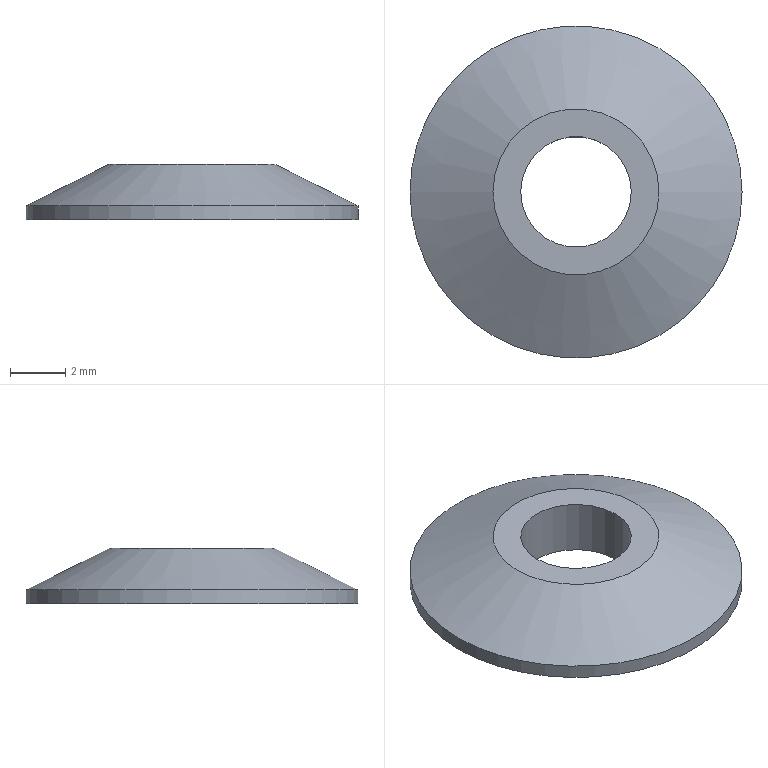Component | NX | 11__27 | 1 solid | 5 faces | box 12 x 12 x 2 mm | volume 130 mm3 | cylinder 2 | plane 2 | cone 1 | commonest cylinder face diameters 4 x1 12 x1
STEP:
#1=CARTESIAN_POINT('',(0.,0.,0.));
#2=DIRECTION('',(0.,0.,1.));
#3=DIRECTION('',(1.,0.,0.));
#4=AXIS2_PLACEMENT_3D('',#1,#2,#3);
#5=CARTESIAN_POINT('',(55.022,109.59,185.932));
#6=VERTEX_POINT('',#5);
#7=CARTESIAN_POINT('',(57.022,109.59,185.932));
#8=DIRECTION('',(0.,0.,-1.));
#9=DIRECTION('',(-1.,0.,0.));
#10=AXIS2_PLACEMENT_3D('',#7,#8,#9);
#11=CIRCLE('',#10,2.);
#12=CARTESIAN_POINT('',(57.022,109.59,187.932));
#13=DIRECTION('',(0.,0.,-1.));
#14=DIRECTION('',(-1.,0.,0.));
#15=AXIS2_PLACEMENT_3D('',#12,#13,#14);
#16=CYLINDRICAL_SURFACE('',#15,2.);
#17=CARTESIAN_POINT('',(0.,2.));
#18=DIRECTION('',(1.,0.));
#19=VECTOR('',#18,1.);
#20=LINE('',#17,#19);
#21=(GEOMETRIC_REPRESENTATION_CONTEXT(2)PARAMETRIC_REPRESENTATION_CONTEXT()REPRESENTATION_CONTEXT('',''));
#22=DEFINITIONAL_REPRESENTATION('',(#20),#21);
#23=PCURVE('',#16,#22);
#24=CARTESIAN_POINT('',(57.022,111.59,185.932));
#25=DIRECTION('',(0.,0.,-1.));
#26=DIRECTION('',(-1.,0.,0.));
#27=AXIS2_PLACEMENT_3D('',#24,#25,#26);
#28=PLANE('',#27);
#29=CARTESIAN_POINT('',(0.,-2.));
#30=DIRECTION('',(1.,0.));
#31=AXIS2_PLACEMENT_2D('',#29,#30);
#32=CIRCLE('',#31,2.);
#33=(GEOMETRIC_REPRESENTATION_CONTEXT(2)PARAMETRIC_REPRESENTATION_CONTEXT()REPRESENTATION_CONTEXT('',''));
#34=DEFINITIONAL_REPRESENTATION('',(#32),#33);
#35=PCURVE('',#28,#34);
#36=SURFACE_CURVE('',#11,(#23,#35),.PCURVE_S1.);
#37=EDGE_CURVE('',#6,#6,#36,.T.);
#38=ORIENTED_EDGE('',*,*,#37,.F.);
#39=CARTESIAN_POINT('',(55.022,109.59,187.932));
#40=VERTEX_POINT('',#39);
#41=CARTESIAN_POINT('',(55.022,109.59,187.932));
#42=CARTESIAN_POINT('',(55.022,109.59,185.932));
#43=B_SPLINE_CURVE_WITH_KNOTS('',1,(#41,#42),.UNSPECIFIED.,.F.,.F.,(2,2),(0.,2.),.PIECEWISE_BEZIER_KNOTS.);
#44=CARTESIAN_POINT('',(0.,0.));
#45=DIRECTION('',(0.,1.));
#46=VECTOR('',#45,1.);
#47=LINE('',#44,#46);
#48=(GEOMETRIC_REPRESENTATION_CONTEXT(2)PARAMETRIC_REPRESENTATION_CONTEXT()REPRESENTATION_CONTEXT('',''));
#49=DEFINITIONAL_REPRESENTATION('',(#47),#48);
#50=PCURVE('',#16,#49);
#51=CARTESIAN_POINT('',(6.283,0.));
#52=DIRECTION('',(0.,1.));
#53=VECTOR('',#52,1.);
#54=LINE('',#51,#53);
#55=(GEOMETRIC_REPRESENTATION_CONTEXT(2)PARAMETRIC_REPRESENTATION_CONTEXT()REPRESENTATION_CONTEXT('',''));
#56=DEFINITIONAL_REPRESENTATION('',(#54),#55);
#57=PCURVE('',#16,#56);
#58=SEAM_CURVE('',#43,(#50,#57),.PCURVE_S1.);
#59=EDGE_CURVE('',#40,#6,#58,.T.);
#60=ORIENTED_EDGE('',*,*,#59,.F.);
#61=CARTESIAN_POINT('',(57.022,109.59,187.932));
#62=DIRECTION('',(0.,0.,-1.));
#63=DIRECTION('',(-1.,0.,0.));
#64=AXIS2_PLACEMENT_3D('',#61,#62,#63);
#65=CIRCLE('',#64,2.);
#66=CARTESIAN_POINT('',(0.,0.));
#67=DIRECTION('',(1.,0.));
#68=VECTOR('',#67,1.);
#69=LINE('',#66,#68);
#70=(GEOMETRIC_REPRESENTATION_CONTEXT(2)PARAMETRIC_REPRESENTATION_CONTEXT()REPRESENTATION_CONTEXT('',''));
#71=DEFINITIONAL_REPRESENTATION('',(#69),#70);
#72=PCURVE('',#16,#71);
#73=CARTESIAN_POINT('',(57.022,112.59,187.932));
#74=DIRECTION('',(0.,0.,1.));
#75=DIRECTION('',(1.,0.,0.));
#76=AXIS2_PLACEMENT_3D('',#73,#74,#75);
#77=PLANE('',#76);
#78=CARTESIAN_POINT('',(-2.,-3.));
#79=CARTESIAN_POINT('',(-2.,0.4641));
#80=CARTESIAN_POINT('',(1.,-1.268));
#81=CARTESIAN_POINT('',(4.,-3.));
#82=CARTESIAN_POINT('',(1.,-4.732));
#83=CARTESIAN_POINT('',(-2.,-6.464));
#84=CARTESIAN_POINT('',(-2.,-3.));
#85=(BOUNDED_CURVE()B_SPLINE_CURVE(2,(#78,#79,#80,#81,#82,#83,#84),.UNSPECIFIED.,.T.,.F.)B_SPLINE_CURVE_WITH_KNOTS((1,2,2,2,2,1),(-2.094,0.,2.094,4.189,6.283,8.378),.UNSPECIFIED.)CURVE()GEOMETRIC_REPRESENTATION_ITEM()RATIONAL_B_SPLINE_CURVE((1.,0.5,1.,0.5,1.,0.5,1.))REPRESENTATION_ITEM(''));
#86=(GEOMETRIC_REPRESENTATION_CONTEXT(2)PARAMETRIC_REPRESENTATION_CONTEXT()REPRESENTATION_CONTEXT('',''));
#87=DEFINITIONAL_REPRESENTATION('',(#85),#86);
#88=PCURVE('',#77,#87);
#89=SURFACE_CURVE('',#65,(#72,#88),.PCURVE_S1.);
#90=EDGE_CURVE('',#40,#40,#89,.T.);
#91=ORIENTED_EDGE('',*,*,#90,.T.);
#92=ORIENTED_EDGE('',*,*,#59,.T.);
#93=EDGE_LOOP('',(#38,#60,#91,#92));
#94=FACE_BOUND('',#93,.F.);
#95=ADVANCED_FACE('',(#94),#16,.F.);
#96=CARTESIAN_POINT('',(51.022,109.59,185.932));
#97=VERTEX_POINT('',#96);
#98=CARTESIAN_POINT('',(57.022,109.59,185.932));
#99=DIRECTION('',(0.,0.,-1.));
#100=DIRECTION('',(-1.,0.,0.));
#101=AXIS2_PLACEMENT_3D('',#98,#99,#100);
#102=CIRCLE('',#101,6.);
#103=CARTESIAN_POINT('',(0.,-2.));
#104=DIRECTION('',(1.,0.));
#105=AXIS2_PLACEMENT_2D('',#103,#104);
#106=CIRCLE('',#105,6.);
#107=(GEOMETRIC_REPRESENTATION_CONTEXT(2)PARAMETRIC_REPRESENTATION_CONTEXT()REPRESENTATION_CONTEXT('',''));
#108=DEFINITIONAL_REPRESENTATION('',(#106),#107);
#109=PCURVE('',#28,#108);
#110=CARTESIAN_POINT('',(57.022,109.59,187.932));
#111=DIRECTION('',(0.,0.,-1.));
#112=DIRECTION('',(-1.,0.,0.));
#113=AXIS2_PLACEMENT_3D('',#110,#111,#112);
#114=CYLINDRICAL_SURFACE('',#113,6.);
#115=CARTESIAN_POINT('',(0.,2.));
#116=DIRECTION('',(1.,0.));
#117=VECTOR('',#116,1.);
#118=LINE('',#115,#117);
#119=(GEOMETRIC_REPRESENTATION_CONTEXT(2)PARAMETRIC_REPRESENTATION_CONTEXT()REPRESENTATION_CONTEXT('',''));
#120=DEFINITIONAL_REPRESENTATION('',(#118),#119);
#121=PCURVE('',#114,#120);
#122=SURFACE_CURVE('',#102,(#109,#121),.PCURVE_S1.);
#123=EDGE_CURVE('',#97,#97,#122,.T.);
#124=ORIENTED_EDGE('',*,*,#123,.T.);
#125=EDGE_LOOP('',(#124));
#126=FACE_BOUND('',#125,.T.);
#127=ORIENTED_EDGE('',*,*,#37,.F.);
#128=EDGE_LOOP('',(#127));
#129=FACE_BOUND('',#128,.T.);
#130=ADVANCED_FACE('',(#126,#129),#28,.T.);
#131=CARTESIAN_POINT('',(51.022,109.59,186.432));
#132=VERTEX_POINT('',#131);
#133=CARTESIAN_POINT('',(57.022,109.59,186.432));
#134=DIRECTION('',(0.,0.,-1.));
#135=DIRECTION('',(-1.,0.,0.));
#136=AXIS2_PLACEMENT_3D('',#133,#134,#135);
#137=CIRCLE('',#136,6.);
#138=CARTESIAN_POINT('',(0.,1.5));
#139=DIRECTION('',(1.,0.));
#140=VECTOR('',#139,1.);
#141=LINE('',#138,#140);
#142=(GEOMETRIC_REPRESENTATION_CONTEXT(2)PARAMETRIC_REPRESENTATION_CONTEXT()REPRESENTATION_CONTEXT('',''));
#143=DEFINITIONAL_REPRESENTATION('',(#141),#142);
#144=PCURVE('',#114,#143);
#145=CARTESIAN_POINT('',(57.022,109.59,186.432));
#146=DIRECTION('',(0.,0.,-1.));
#147=DIRECTION('',(-1.,0.,0.));
#148=AXIS2_PLACEMENT_3D('',#145,#146,#147);
#149=CONICAL_SURFACE('',#148,6.,1.107);
#150=CARTESIAN_POINT('',(0.,0.));
#151=DIRECTION('',(1.,0.));
#152=VECTOR('',#151,1.);
#153=LINE('',#150,#152);
#154=(GEOMETRIC_REPRESENTATION_CONTEXT(2)PARAMETRIC_REPRESENTATION_CONTEXT()REPRESENTATION_CONTEXT('',''));
#155=DEFINITIONAL_REPRESENTATION('',(#153),#154);
#156=PCURVE('',#149,#155);
#157=SURFACE_CURVE('',#137,(#144,#156),.PCURVE_S1.);
#158=EDGE_CURVE('',#132,#132,#157,.T.);
#159=ORIENTED_EDGE('',*,*,#158,.T.);
#160=CARTESIAN_POINT('',(51.022,109.59,186.432));
#161=CARTESIAN_POINT('',(51.022,109.59,185.932));
#162=B_SPLINE_CURVE_WITH_KNOTS('',1,(#160,#161),.UNSPECIFIED.,.F.,.F.,(2,2),(1.5,2.),.PIECEWISE_BEZIER_KNOTS.);
#163=CARTESIAN_POINT('',(6.283,0.));
#164=DIRECTION('',(0.,1.));
#165=VECTOR('',#164,1.);
#166=LINE('',#163,#165);
#167=(GEOMETRIC_REPRESENTATION_CONTEXT(2)PARAMETRIC_REPRESENTATION_CONTEXT()REPRESENTATION_CONTEXT('',''));
#168=DEFINITIONAL_REPRESENTATION('',(#166),#167);
#169=PCURVE('',#114,#168);
#170=CARTESIAN_POINT('',(0.,0.));
#171=DIRECTION('',(0.,1.));
#172=VECTOR('',#171,1.);
#173=LINE('',#170,#172);
#174=(GEOMETRIC_REPRESENTATION_CONTEXT(2)PARAMETRIC_REPRESENTATION_CONTEXT()REPRESENTATION_CONTEXT('',''));
#175=DEFINITIONAL_REPRESENTATION('',(#173),#174);
#176=PCURVE('',#114,#175);
#177=SEAM_CURVE('',#162,(#169,#176),.PCURVE_S1.);
#178=EDGE_CURVE('',#132,#97,#177,.T.);
#179=ORIENTED_EDGE('',*,*,#178,.T.);
#180=ORIENTED_EDGE('',*,*,#123,.F.);
#181=ORIENTED_EDGE('',*,*,#178,.F.);
#182=EDGE_LOOP('',(#159,#179,#180,#181));
#183=FACE_BOUND('',#182,.T.);
#184=ADVANCED_FACE('',(#183),#114,.T.);
#185=CARTESIAN_POINT('',(54.022,109.59,187.932));
#186=VERTEX_POINT('',#185);
#187=CARTESIAN_POINT('',(57.022,109.59,187.932));
#188=DIRECTION('',(0.,0.,-1.));
#189=DIRECTION('',(-1.,0.,0.));
#190=AXIS2_PLACEMENT_3D('',#187,#188,#189);
#191=CIRCLE('',#190,3.);
#192=CARTESIAN_POINT('',(0.,-1.5));
#193=DIRECTION('',(1.,0.));
#194=VECTOR('',#193,1.);
#195=LINE('',#192,#194);
#196=(GEOMETRIC_REPRESENTATION_CONTEXT(2)PARAMETRIC_REPRESENTATION_CONTEXT()REPRESENTATION_CONTEXT('',''));
#197=DEFINITIONAL_REPRESENTATION('',(#195),#196);
#198=PCURVE('',#149,#197);
#199=CARTESIAN_POINT('',(-3.,-3.));
#200=CARTESIAN_POINT('',(-3.,2.196));
#201=CARTESIAN_POINT('',(1.5,-0.4019));
#202=CARTESIAN_POINT('',(6.,-3.));
#203=CARTESIAN_POINT('',(1.5,-5.598));
#204=CARTESIAN_POINT('',(-3.,-8.196));
#205=CARTESIAN_POINT('',(-3.,-3.));
#206=(BOUNDED_CURVE()B_SPLINE_CURVE(2,(#199,#200,#201,#202,#203,#204,#205),.UNSPECIFIED.,.T.,.F.)B_SPLINE_CURVE_WITH_KNOTS((1,2,2,2,2,1),(-2.094,0.,2.094,4.189,6.283,8.378),.UNSPECIFIED.)CURVE()GEOMETRIC_REPRESENTATION_ITEM()RATIONAL_B_SPLINE_CURVE((1.,0.5,1.,0.5,1.,0.5,1.))REPRESENTATION_ITEM(''));
#207=(GEOMETRIC_REPRESENTATION_CONTEXT(2)PARAMETRIC_REPRESENTATION_CONTEXT()REPRESENTATION_CONTEXT('',''));
#208=DEFINITIONAL_REPRESENTATION('',(#206),#207);
#209=PCURVE('',#77,#208);
#210=SURFACE_CURVE('',#191,(#198,#209),.PCURVE_S1.);
#211=EDGE_CURVE('',#186,#186,#210,.T.);
#212=ORIENTED_EDGE('',*,*,#211,.T.);
#213=CARTESIAN_POINT('',(54.022,109.59,187.932));
#214=CARTESIAN_POINT('',(51.022,109.59,186.432));
#215=B_SPLINE_CURVE_WITH_KNOTS('',1,(#213,#214),.UNSPECIFIED.,.F.,.F.,(2,2),(-3.354,0.),.PIECEWISE_BEZIER_KNOTS.);
#216=CARTESIAN_POINT('',(6.283,0.));
#217=DIRECTION('',(0.,1.));
#218=VECTOR('',#217,1.);
#219=LINE('',#216,#218);
#220=(GEOMETRIC_REPRESENTATION_CONTEXT(2)PARAMETRIC_REPRESENTATION_CONTEXT()REPRESENTATION_CONTEXT('',''));
#221=DEFINITIONAL_REPRESENTATION('',(#219),#220);
#222=PCURVE('',#149,#221);
#223=CARTESIAN_POINT('',(0.,0.));
#224=DIRECTION('',(0.,1.));
#225=VECTOR('',#224,1.);
#226=LINE('',#223,#225);
#227=(GEOMETRIC_REPRESENTATION_CONTEXT(2)PARAMETRIC_REPRESENTATION_CONTEXT()REPRESENTATION_CONTEXT('',''));
#228=DEFINITIONAL_REPRESENTATION('',(#226),#227);
#229=PCURVE('',#149,#228);
#230=SEAM_CURVE('',#215,(#222,#229),.PCURVE_S1.);
#231=EDGE_CURVE('',#186,#132,#230,.T.);
#232=ORIENTED_EDGE('',*,*,#231,.T.);
#233=ORIENTED_EDGE('',*,*,#158,.F.);
#234=ORIENTED_EDGE('',*,*,#231,.F.);
#235=EDGE_LOOP('',(#212,#232,#233,#234));
#236=FACE_BOUND('',#235,.T.);
#237=ADVANCED_FACE('',(#236),#149,.T.);
#238=ORIENTED_EDGE('',*,*,#90,.T.);
#239=EDGE_LOOP('',(#238));
#240=FACE_BOUND('',#239,.T.);
#241=ORIENTED_EDGE('',*,*,#211,.F.);
#242=EDGE_LOOP('',(#241));
#243=FACE_BOUND('',#242,.T.);
#244=ADVANCED_FACE('',(#240,#243),#77,.T.);
#245=CLOSED_SHELL('',(#95,#130,#184,#237,#244));
#246=MANIFOLD_SOLID_BREP('',#245);
#247=(LENGTH_UNIT()NAMED_UNIT(*)SI_UNIT(.MILLI.,.METRE.));
#248=UNCERTAINTY_MEASURE_WITH_UNIT(LENGTH_MEASURE(0.00001),#247,'','');
#249=(NAMED_UNIT(*)PLANE_ANGLE_UNIT()SI_UNIT($,.RADIAN.));
#250=(NAMED_UNIT(*)SI_UNIT($,.STERADIAN.)SOLID_ANGLE_UNIT());
#251=(GEOMETRIC_REPRESENTATION_CONTEXT(3)GLOBAL_UNCERTAINTY_ASSIGNED_CONTEXT((#248))GLOBAL_UNIT_ASSIGNED_CONTEXT((#247,#249,#250))REPRESENTATION_CONTEXT('',''));
#252=ADVANCED_BREP_SHAPE_REPRESENTATION('',(#4,#246),#251);